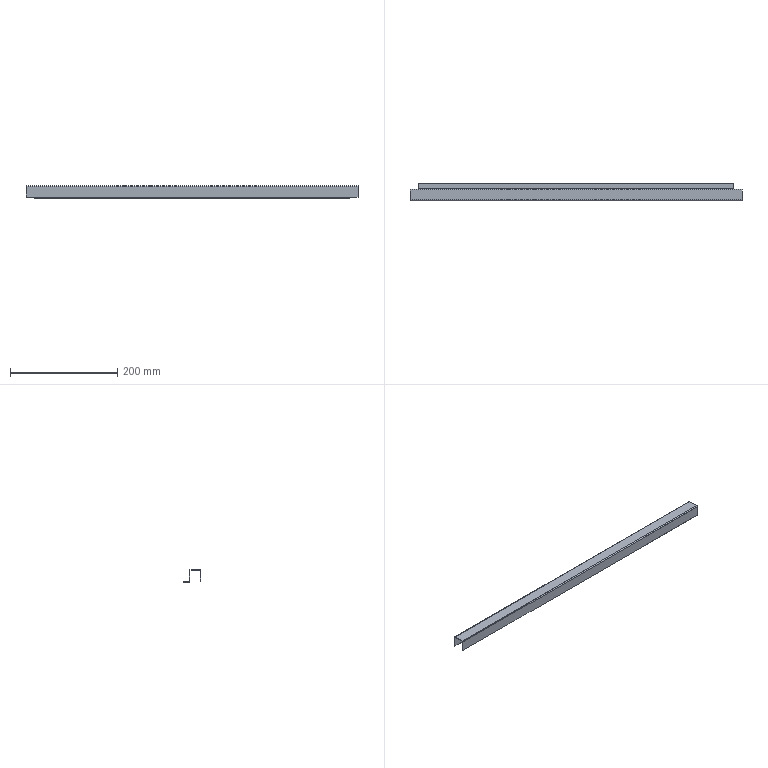Component | SolidWorks | CCQ-1.1-17LowerBeam1-1 | 1 solid | 34 faces | box 620 x 33 x 23 mm | volume 45090 mm3 | plane 24 | cylinder 10 | commonest cylinder face diameters 6 x4 1.473 x3 3.473 x3 | material 304
STEP:
#1=CARTESIAN_POINT('',(-0.2756,-17.185,0.7087));
#2=VERTEX_POINT('',#1);
#3=CARTESIAN_POINT('',(-0.2756,-17.185,0.4724));
#4=VERTEX_POINT('',#3);
#5=CARTESIAN_POINT('',(-0.2756,-17.185,0.5906));
#6=DIRECTION('',(0.,-1.,0.));
#7=DIRECTION('',(0.,0.,-1.));
#8=AXIS2_PLACEMENT_3D('',#5,#6,#7);
#9=CIRCLE('',#8,0.1181);
#10=EDGE_CURVE('',#2,#4,#9,.T.);
#11=ORIENTED_EDGE('',*,*,#10,.T.);
#12=CARTESIAN_POINT('',(-0.2756,-17.146,0.4724));
#13=VERTEX_POINT('',#12);
#14=CARTESIAN_POINT('',(-0.2756,-17.539,0.4724));
#15=DIRECTION('',(0.,1.,0.));
#16=VECTOR('',#15,39.37);
#17=LINE('',#14,#16);
#18=EDGE_CURVE('',#4,#13,#17,.T.);
#19=ORIENTED_EDGE('',*,*,#18,.T.);
#20=CARTESIAN_POINT('',(-0.2756,-17.146,0.7087));
#21=VERTEX_POINT('',#20);
#22=CARTESIAN_POINT('',(-0.2756,-17.146,0.5906));
#23=DIRECTION('',(0.,1.,0.));
#24=DIRECTION('',(0.,0.,-1.));
#25=AXIS2_PLACEMENT_3D('',#22,#23,#24);
#26=CIRCLE('',#25,0.1181);
#27=EDGE_CURVE('',#13,#21,#26,.T.);
#28=ORIENTED_EDGE('',*,*,#27,.T.);
#29=CARTESIAN_POINT('',(-0.2756,-17.539,0.7087));
#30=DIRECTION('',(0.,1.,0.));
#31=VECTOR('',#30,39.37);
#32=LINE('',#29,#31);
#33=EDGE_CURVE('',#2,#21,#32,.T.);
#34=ORIENTED_EDGE('',*,*,#33,.F.);
#35=EDGE_LOOP('',(#11,#19,#28,#34));
#36=FACE_OUTER_BOUND('',#35,.T.);
#37=CARTESIAN_POINT('',(-0.2756,-17.539,0.5906));
#38=DIRECTION('',(0.,1.,0.));
#39=DIRECTION('',(0.,0.,1.));
#40=AXIS2_PLACEMENT_3D('',#37,#38,#39);
#41=CYLINDRICAL_SURFACE('',#40,0.1181);
#42=ADVANCED_FACE('',(#36),#41,.F.);
#43=CARTESIAN_POINT('',(-24.134,-17.185,0.7087));
#44=VERTEX_POINT('',#43);
#45=CARTESIAN_POINT('',(-24.134,-17.185,0.4724));
#46=VERTEX_POINT('',#45);
#47=CARTESIAN_POINT('',(-24.134,-17.185,0.5906));
#48=DIRECTION('',(0.,-1.,0.));
#49=DIRECTION('',(0.,0.,-1.));
#50=AXIS2_PLACEMENT_3D('',#47,#48,#49);
#51=CIRCLE('',#50,0.1181);
#52=EDGE_CURVE('',#44,#46,#51,.T.);
#53=ORIENTED_EDGE('',*,*,#52,.T.);
#54=CARTESIAN_POINT('',(-24.134,-17.146,0.4724));
#55=VERTEX_POINT('',#54);
#56=CARTESIAN_POINT('',(-24.134,-17.539,0.4724));
#57=DIRECTION('',(0.,1.,0.));
#58=VECTOR('',#57,39.37);
#59=LINE('',#56,#58);
#60=EDGE_CURVE('',#46,#55,#59,.T.);
#61=ORIENTED_EDGE('',*,*,#60,.T.);
#62=CARTESIAN_POINT('',(-24.134,-17.146,0.7087));
#63=VERTEX_POINT('',#62);
#64=CARTESIAN_POINT('',(-24.134,-17.146,0.5906));
#65=DIRECTION('',(0.,1.,0.));
#66=DIRECTION('',(0.,0.,1.));
#67=AXIS2_PLACEMENT_3D('',#64,#65,#66);
#68=CIRCLE('',#67,0.1181);
#69=EDGE_CURVE('',#55,#63,#68,.T.);
#70=ORIENTED_EDGE('',*,*,#69,.T.);
#71=CARTESIAN_POINT('',(-24.134,-17.539,0.7087));
#72=DIRECTION('',(0.,1.,0.));
#73=VECTOR('',#72,39.37);
#74=LINE('',#71,#73);
#75=EDGE_CURVE('',#44,#63,#74,.T.);
#76=ORIENTED_EDGE('',*,*,#75,.F.);
#77=EDGE_LOOP('',(#53,#61,#70,#76));
#78=FACE_OUTER_BOUND('',#77,.T.);
#79=CARTESIAN_POINT('',(-24.134,-17.539,0.5906));
#80=DIRECTION('',(0.,1.,0.));
#81=DIRECTION('',(0.,0.,1.));
#82=AXIS2_PLACEMENT_3D('',#79,#80,#81);
#83=CYLINDRICAL_SURFACE('',#82,0.1181);
#84=ADVANCED_FACE('',(#78),#83,.F.);
#85=CARTESIAN_POINT('',(0.,-17.146,-0.04961));
#86=VERTEX_POINT('',#85);
#87=CARTESIAN_POINT('',(0.,-17.185,-0.04961));
#88=VERTEX_POINT('',#87);
#89=CARTESIAN_POINT('',(0.,-17.117,-0.04961));
#90=DIRECTION('',(0.,-1.,0.));
#91=VECTOR('',#90,39.37);
#92=LINE('',#89,#91);
#93=EDGE_CURVE('',#86,#88,#92,.T.);
#94=ORIENTED_EDGE('',*,*,#93,.F.);
#95=CARTESIAN_POINT('',(0.,-17.146,0.719));
#96=VERTEX_POINT('',#95);
#97=CARTESIAN_POINT('',(0.,-17.146,0.748));
#98=DIRECTION('',(0.,0.,1.));
#99=VECTOR('',#98,39.37);
#100=LINE('',#97,#99);
#101=EDGE_CURVE('',#86,#96,#100,.T.);
#102=ORIENTED_EDGE('',*,*,#101,.T.);
#103=CARTESIAN_POINT('',(0.,-17.185,0.719));
#104=VERTEX_POINT('',#103);
#105=CARTESIAN_POINT('',(0.,-17.146,0.719));
#106=DIRECTION('',(0.,-1.,0.));
#107=VECTOR('',#106,39.37);
#108=LINE('',#105,#107);
#109=EDGE_CURVE('',#96,#104,#108,.T.);
#110=ORIENTED_EDGE('',*,*,#109,.T.);
#111=CARTESIAN_POINT('',(0.,-17.185,0.748));
#112=DIRECTION('',(0.,0.,1.));
#113=VECTOR('',#112,39.37);
#114=LINE('',#111,#113);
#115=EDGE_CURVE('',#88,#104,#114,.T.);
#116=ORIENTED_EDGE('',*,*,#115,.F.);
#117=EDGE_LOOP('',(#94,#102,#110,#116));
#118=FACE_OUTER_BOUND('',#117,.T.);
#119=CARTESIAN_POINT('',(0.,-17.117,-0.07874));
#120=DIRECTION('',(1.,0.,0.));
#121=DIRECTION('',(0.,0.,-1.));
#122=AXIS2_PLACEMENT_3D('',#119,#120,#121);
#123=PLANE('',#122);
#124=ADVANCED_FACE('',(#118),#123,.T.);
#125=CARTESIAN_POINT('',(0.,-17.214,0.748));
#126=VERTEX_POINT('',#125);
#127=CARTESIAN_POINT('',(0.,-17.214,0.7874));
#128=VERTEX_POINT('',#127);
#129=CARTESIAN_POINT('',(0.,-17.214,0.748));
#130=DIRECTION('',(0.,0.,1.));
#131=VECTOR('',#130,39.37);
#132=LINE('',#129,#131);
#133=EDGE_CURVE('',#126,#128,#132,.T.);
#134=ORIENTED_EDGE('',*,*,#133,.F.);
#135=CARTESIAN_POINT('',(0.,-17.214,0.719));
#136=DIRECTION('',(1.,0.,0.));
#137=DIRECTION('',(0.,0.,1.));
#138=AXIS2_PLACEMENT_3D('',#135,#136,#137);
#139=CIRCLE('',#138,0.029);
#140=EDGE_CURVE('',#104,#126,#139,.T.);
#141=ORIENTED_EDGE('',*,*,#140,.F.);
#142=ORIENTED_EDGE('',*,*,#109,.F.);
#143=CARTESIAN_POINT('',(0.,-17.214,0.719));
#144=DIRECTION('',(1.,0.,0.));
#145=DIRECTION('',(0.,0.,-1.));
#146=AXIS2_PLACEMENT_3D('',#143,#144,#145);
#147=CIRCLE('',#146,0.06837);
#148=EDGE_CURVE('',#96,#128,#147,.T.);
#149=ORIENTED_EDGE('',*,*,#148,.T.);
#150=EDGE_LOOP('',(#134,#141,#142,#149));
#151=FACE_OUTER_BOUND('',#150,.T.);
#152=CARTESIAN_POINT('',(0.,-17.214,0.748));
#153=DIRECTION('',(1.,0.,0.));
#154=DIRECTION('',(0.,0.,-1.));
#155=AXIS2_PLACEMENT_3D('',#152,#153,#154);
#156=PLANE('',#155);
#157=ADVANCED_FACE('',(#151),#156,.T.);
#158=CARTESIAN_POINT('',(0.,-17.943,0.748));
#159=VERTEX_POINT('',#158);
#160=CARTESIAN_POINT('',(0.,-17.972,0.748));
#161=DIRECTION('',(0.,-1.,0.));
#162=VECTOR('',#161,39.37);
#163=LINE('',#160,#162);
#164=EDGE_CURVE('',#126,#159,#163,.T.);
#165=ORIENTED_EDGE('',*,*,#164,.F.);
#166=ORIENTED_EDGE('',*,*,#133,.T.);
#167=CARTESIAN_POINT('',(0.,-17.943,0.7874));
#168=VERTEX_POINT('',#167);
#169=CARTESIAN_POINT('',(0.,-17.972,0.7874));
#170=DIRECTION('',(0.,-1.,0.));
#171=VECTOR('',#170,39.37);
#172=LINE('',#169,#171);
#173=EDGE_CURVE('',#128,#168,#172,.T.);
#174=ORIENTED_EDGE('',*,*,#173,.T.);
#175=CARTESIAN_POINT('',(0.,-17.943,0.7874));
#176=DIRECTION('',(0.,-0.,-1.));
#177=VECTOR('',#176,39.37);
#178=LINE('',#175,#177);
#179=EDGE_CURVE('',#168,#159,#178,.T.);
#180=ORIENTED_EDGE('',*,*,#179,.T.);
#181=EDGE_LOOP('',(#165,#166,#174,#180));
#182=FACE_OUTER_BOUND('',#181,.T.);
#183=CARTESIAN_POINT('',(0.,-17.146,0.719));
#184=DIRECTION('',(1.,0.,0.));
#185=DIRECTION('',(0.,0.,-1.));
#186=AXIS2_PLACEMENT_3D('',#183,#184,#185);
#187=PLANE('',#186);
#188=ADVANCED_FACE('',(#182),#187,.T.);
#189=CARTESIAN_POINT('',(-24.409,-17.185,0.719));
#190=VERTEX_POINT('',#189);
#191=CARTESIAN_POINT('',(-24.409,-17.146,0.719));
#192=VERTEX_POINT('',#191);
#193=CARTESIAN_POINT('',(-24.409,-17.185,0.719));
#194=DIRECTION('',(0.,1.,-0.));
#195=VECTOR('',#194,39.37);
#196=LINE('',#193,#195);
#197=EDGE_CURVE('',#190,#192,#196,.T.);
#198=ORIENTED_EDGE('',*,*,#197,.F.);
#199=CARTESIAN_POINT('',(-24.409,-17.214,0.748));
#200=VERTEX_POINT('',#199);
#201=CARTESIAN_POINT('',(-24.409,-17.214,0.719));
#202=DIRECTION('',(1.,0.,0.));
#203=DIRECTION('',(0.,0.,1.));
#204=AXIS2_PLACEMENT_3D('',#201,#202,#203);
#205=CIRCLE('',#204,0.029);
#206=EDGE_CURVE('',#190,#200,#205,.T.);
#207=ORIENTED_EDGE('',*,*,#206,.T.);
#208=CARTESIAN_POINT('',(-24.409,-17.214,0.7874));
#209=VERTEX_POINT('',#208);
#210=CARTESIAN_POINT('',(-24.409,-17.214,0.7874));
#211=DIRECTION('',(0.,0.,-1.));
#212=VECTOR('',#211,39.37);
#213=LINE('',#210,#212);
#214=EDGE_CURVE('',#209,#200,#213,.T.);
#215=ORIENTED_EDGE('',*,*,#214,.F.);
#216=CARTESIAN_POINT('',(-24.409,-17.214,0.719));
#217=DIRECTION('',(1.,0.,0.));
#218=DIRECTION('',(0.,0.,-1.));
#219=AXIS2_PLACEMENT_3D('',#216,#217,#218);
#220=CIRCLE('',#219,0.06837);
#221=EDGE_CURVE('',#192,#209,#220,.T.);
#222=ORIENTED_EDGE('',*,*,#221,.F.);
#223=EDGE_LOOP('',(#198,#207,#215,#222));
#224=FACE_OUTER_BOUND('',#223,.T.);
#225=CARTESIAN_POINT('',(-24.409,-17.185,0.719));
#226=DIRECTION('',(-1.,0.,0.));
#227=DIRECTION('',(0.,0.,1.));
#228=AXIS2_PLACEMENT_3D('',#225,#226,#227);
#229=PLANE('',#228);
#230=ADVANCED_FACE('',(#224),#229,.T.);
#231=CARTESIAN_POINT('',(-24.409,-17.185,-0.04961));
#232=VERTEX_POINT('',#231);
#233=CARTESIAN_POINT('',(-24.409,-17.146,-0.04961));
#234=VERTEX_POINT('',#233);
#235=CARTESIAN_POINT('',(-24.409,-17.214,-0.04961));
#236=DIRECTION('',(0.,1.,0.));
#237=VECTOR('',#236,39.37);
#238=LINE('',#235,#237);
#239=EDGE_CURVE('',#232,#234,#238,.T.);
#240=ORIENTED_EDGE('',*,*,#239,.F.);
#241=CARTESIAN_POINT('',(-24.409,-17.185,0.748));
#242=DIRECTION('',(0.,0.,1.));
#243=VECTOR('',#242,39.37);
#244=LINE('',#241,#243);
#245=EDGE_CURVE('',#232,#190,#244,.T.);
#246=ORIENTED_EDGE('',*,*,#245,.T.);
#247=ORIENTED_EDGE('',*,*,#197,.T.);
#248=CARTESIAN_POINT('',(-24.409,-17.146,0.748));
#249=DIRECTION('',(0.,0.,1.));
#250=VECTOR('',#249,39.37);
#251=LINE('',#248,#250);
#252=EDGE_CURVE('',#234,#192,#251,.T.);
#253=ORIENTED_EDGE('',*,*,#252,.F.);
#254=EDGE_LOOP('',(#240,#246,#247,#253));
#255=FACE_OUTER_BOUND('',#254,.T.);
#256=CARTESIAN_POINT('',(-24.409,-17.214,0.7874));
#257=DIRECTION('',(-1.,0.,0.));
#258=DIRECTION('',(0.,0.,1.));
#259=AXIS2_PLACEMENT_3D('',#256,#257,#258);
#260=PLANE('',#259);
#261=ADVANCED_FACE('',(#255),#260,.T.);
#262=CARTESIAN_POINT('',(0.,-17.972,0.719));
#263=VERTEX_POINT('',#262);
#264=CARTESIAN_POINT('',(0.,-18.012,0.719));
#265=VERTEX_POINT('',#264);
#266=CARTESIAN_POINT('',(0.,-17.972,0.719));
#267=DIRECTION('',(0.,-1.,0.));
#268=VECTOR('',#267,39.37);
#269=LINE('',#266,#268);
#270=EDGE_CURVE('',#263,#265,#269,.T.);
#271=ORIENTED_EDGE('',*,*,#270,.F.);
#272=CARTESIAN_POINT('',(0.,-17.943,0.719));
#273=DIRECTION('',(1.,0.,0.));
#274=DIRECTION('',(0.,0.,1.));
#275=AXIS2_PLACEMENT_3D('',#272,#273,#274);
#276=CIRCLE('',#275,0.029);
#277=EDGE_CURVE('',#159,#263,#276,.T.);
#278=ORIENTED_EDGE('',*,*,#277,.F.);
#279=ORIENTED_EDGE('',*,*,#179,.F.);
#280=CARTESIAN_POINT('',(0.,-17.943,0.719));
#281=DIRECTION('',(1.,0.,0.));
#282=DIRECTION('',(0.,0.,-1.));
#283=AXIS2_PLACEMENT_3D('',#280,#281,#282);
#284=CIRCLE('',#283,0.06837);
#285=EDGE_CURVE('',#168,#265,#284,.T.);
#286=ORIENTED_EDGE('',*,*,#285,.T.);
#287=EDGE_LOOP('',(#271,#278,#279,#286));
#288=FACE_OUTER_BOUND('',#287,.T.);
#289=CARTESIAN_POINT('',(0.,-17.972,0.719));
#290=DIRECTION('',(1.,0.,0.));
#291=DIRECTION('',(0.,0.,-1.));
#292=AXIS2_PLACEMENT_3D('',#289,#290,#291);
#293=PLANE('',#292);
#294=ADVANCED_FACE('',(#288),#293,.T.);
#295=CARTESIAN_POINT('',(0.,-17.972,-0.03937));
#296=VERTEX_POINT('',#295);
#297=CARTESIAN_POINT('',(0.,-17.972,0.748));
#298=DIRECTION('',(0.,0.,-1.));
#299=VECTOR('',#298,39.37);
#300=LINE('',#297,#299);
#301=EDGE_CURVE('',#263,#296,#300,.T.);
#302=ORIENTED_EDGE('',*,*,#301,.F.);
#303=ORIENTED_EDGE('',*,*,#270,.T.);
#304=CARTESIAN_POINT('',(0.,-18.012,-0.03937));
#305=VERTEX_POINT('',#304);
#306=CARTESIAN_POINT('',(0.,-18.012,0.748));
#307=DIRECTION('',(0.,0.,-1.));
#308=VECTOR('',#307,39.37);
#309=LINE('',#306,#308);
#310=EDGE_CURVE('',#265,#305,#309,.T.);
#311=ORIENTED_EDGE('',*,*,#310,.T.);
#312=CARTESIAN_POINT('',(0.,-17.972,-0.03937));
#313=DIRECTION('',(0.,-1.,0.));
#314=VECTOR('',#313,39.37);
#315=LINE('',#312,#314);
#316=EDGE_CURVE('',#296,#305,#315,.T.);
#317=ORIENTED_EDGE('',*,*,#316,.F.);
#318=EDGE_LOOP('',(#302,#303,#311,#317));
#319=FACE_OUTER_BOUND('',#318,.T.);
#320=CARTESIAN_POINT('',(0.,-17.943,0.7874));
#321=DIRECTION('',(1.,0.,0.));
#322=DIRECTION('',(0.,0.,-1.));
#323=AXIS2_PLACEMENT_3D('',#320,#321,#322);
#324=PLANE('',#323);
#325=ADVANCED_FACE('',(#319),#324,.T.);
#326=CARTESIAN_POINT('',(-24.409,-17.943,0.748));
#327=VERTEX_POINT('',#326);
#328=CARTESIAN_POINT('',(-24.409,-17.943,0.7874));
#329=VERTEX_POINT('',#328);
#330=CARTESIAN_POINT('',(-24.409,-17.943,0.748));
#331=DIRECTION('',(0.,0.,1.));
#332=VECTOR('',#331,39.37);
#333=LINE('',#330,#332);
#334=EDGE_CURVE('',#327,#329,#333,.T.);
#335=ORIENTED_EDGE('',*,*,#334,.F.);
#336=CARTESIAN_POINT('',(-24.409,-17.972,0.719));
#337=VERTEX_POINT('',#336);
#338=CARTESIAN_POINT('',(-24.409,-17.943,0.719));
#339=DIRECTION('',(1.,0.,0.));
#340=DIRECTION('',(0.,0.,1.));
#341=AXIS2_PLACEMENT_3D('',#338,#339,#340);
#342=CIRCLE('',#341,0.029);
#343=EDGE_CURVE('',#327,#337,#342,.T.);
#344=ORIENTED_EDGE('',*,*,#343,.T.);
#345=CARTESIAN_POINT('',(-24.409,-18.012,0.719));
#346=VERTEX_POINT('',#345);
#347=CARTESIAN_POINT('',(-24.409,-18.012,0.719));
#348=DIRECTION('',(0.,1.,0.));
#349=VECTOR('',#348,39.37);
#350=LINE('',#347,#349);
#351=EDGE_CURVE('',#346,#337,#350,.T.);
#352=ORIENTED_EDGE('',*,*,#351,.F.);
#353=CARTESIAN_POINT('',(-24.409,-17.943,0.719));
#354=DIRECTION('',(1.,0.,0.));
#355=DIRECTION('',(0.,0.,-1.));
#356=AXIS2_PLACEMENT_3D('',#353,#354,#355);
#357=CIRCLE('',#356,0.06837);
#358=EDGE_CURVE('',#329,#346,#357,.T.);
#359=ORIENTED_EDGE('',*,*,#358,.F.);
#360=EDGE_LOOP('',(#335,#344,#352,#359));
#361=FACE_OUTER_BOUND('',#360,.T.);
#362=CARTESIAN_POINT('',(-24.409,-17.943,0.748));
#363=DIRECTION('',(-1.,0.,0.));
#364=DIRECTION('',(0.,0.,1.));
#365=AXIS2_PLACEMENT_3D('',#362,#363,#364);
#366=PLANE('',#365);
#367=ADVANCED_FACE('',(#361),#366,.T.);
#368=CARTESIAN_POINT('',(-24.409,-17.972,0.748));
#369=DIRECTION('',(0.,-1.,0.));
#370=VECTOR('',#369,39.37);
#371=LINE('',#368,#370);
#372=EDGE_CURVE('',#200,#327,#371,.T.);
#373=ORIENTED_EDGE('',*,*,#372,.T.);
#374=ORIENTED_EDGE('',*,*,#334,.T.);
#375=CARTESIAN_POINT('',(-24.409,-17.972,0.7874));
#376=DIRECTION('',(0.,-1.,0.));
#377=VECTOR('',#376,39.37);
#378=LINE('',#375,#377);
#379=EDGE_CURVE('',#209,#329,#378,.T.);
#380=ORIENTED_EDGE('',*,*,#379,.F.);
#381=ORIENTED_EDGE('',*,*,#214,.T.);
#382=EDGE_LOOP('',(#373,#374,#380,#381));
#383=FACE_OUTER_BOUND('',#382,.T.);
#384=CARTESIAN_POINT('',(-24.409,-18.012,0.719));
#385=DIRECTION('',(-1.,0.,0.));
#386=DIRECTION('',(0.,0.,1.));
#387=AXIS2_PLACEMENT_3D('',#384,#385,#386);
#388=PLANE('',#387);
#389=ADVANCED_FACE('',(#383),#388,.T.);
#390=CARTESIAN_POINT('',(-24.409,-18.012,-0.03937));
#391=VERTEX_POINT('',#390);
#392=CARTESIAN_POINT('',(-24.409,-18.012,0.748));
#393=DIRECTION('',(0.,0.,-1.));
#394=VECTOR('',#393,39.37);
#395=LINE('',#392,#394);
#396=EDGE_CURVE('',#346,#391,#395,.T.);
#397=ORIENTED_EDGE('',*,*,#396,.T.);
#398=CARTESIAN_POINT('',(0.,-18.012,-0.03937));
#399=DIRECTION('',(-1.,0.,0.));
#400=VECTOR('',#399,39.37);
#401=LINE('',#398,#400);
#402=EDGE_CURVE('',#305,#391,#401,.T.);
#403=ORIENTED_EDGE('',*,*,#402,.F.);
#404=ORIENTED_EDGE('',*,*,#310,.F.);
#405=CARTESIAN_POINT('',(0.,-18.012,0.719));
#406=DIRECTION('',(-1.,0.,0.));
#407=VECTOR('',#406,39.37);
#408=LINE('',#405,#407);
#409=EDGE_CURVE('',#265,#346,#408,.T.);
#410=ORIENTED_EDGE('',*,*,#409,.T.);
#411=EDGE_LOOP('',(#397,#403,#404,#410));
#412=FACE_OUTER_BOUND('',#411,.T.);
#413=CARTESIAN_POINT('',(0.,-18.012,0.748));
#414=DIRECTION('',(0.,1.,0.));
#415=DIRECTION('',(0.,0.,1.));
#416=AXIS2_PLACEMENT_3D('',#413,#414,#415);
#417=PLANE('',#416);
#418=ADVANCED_FACE('',(#412),#417,.F.);
#419=CARTESIAN_POINT('',(-24.409,-17.972,-0.03937));
#420=VERTEX_POINT('',#419);
#421=CARTESIAN_POINT('',(-24.409,-17.972,-0.03937));
#422=DIRECTION('',(0.,-1.,0.));
#423=VECTOR('',#422,39.37);
#424=LINE('',#421,#423);
#425=EDGE_CURVE('',#420,#391,#424,.T.);
#426=ORIENTED_EDGE('',*,*,#425,.F.);
#427=CARTESIAN_POINT('',(0.,-17.972,-0.03937));
#428=DIRECTION('',(-1.,0.,0.));
#429=VECTOR('',#428,39.37);
#430=LINE('',#427,#429);
#431=EDGE_CURVE('',#296,#420,#430,.T.);
#432=ORIENTED_EDGE('',*,*,#431,.F.);
#433=ORIENTED_EDGE('',*,*,#316,.T.);
#434=ORIENTED_EDGE('',*,*,#402,.T.);
#435=EDGE_LOOP('',(#426,#432,#433,#434));
#436=FACE_OUTER_BOUND('',#435,.T.);
#437=CARTESIAN_POINT('',(0.,-17.972,-0.03937));
#438=DIRECTION('',(0.,0.,-1.));
#439=DIRECTION('',(-1.,0.,0.));
#440=AXIS2_PLACEMENT_3D('',#437,#438,#439);
#441=PLANE('',#440);
#442=ADVANCED_FACE('',(#436),#441,.T.);
#443=CARTESIAN_POINT('',(-24.409,-17.972,0.748));
#444=DIRECTION('',(0.,0.,-1.));
#445=VECTOR('',#444,39.37);
#446=LINE('',#443,#445);
#447=EDGE_CURVE('',#337,#420,#446,.T.);
#448=ORIENTED_EDGE('',*,*,#447,.F.);
#449=CARTESIAN_POINT('',(0.,-17.972,0.719));
#450=DIRECTION('',(-1.,0.,0.));
#451=VECTOR('',#450,39.37);
#452=LINE('',#449,#451);
#453=EDGE_CURVE('',#263,#337,#452,.T.);
#454=ORIENTED_EDGE('',*,*,#453,.F.);
#455=ORIENTED_EDGE('',*,*,#301,.T.);
#456=ORIENTED_EDGE('',*,*,#431,.T.);
#457=EDGE_LOOP('',(#448,#454,#455,#456));
#458=FACE_OUTER_BOUND('',#457,.T.);
#459=CARTESIAN_POINT('',(0.,-17.972,0.748));
#460=DIRECTION('',(0.,1.,0.));
#461=DIRECTION('',(0.,0.,1.));
#462=AXIS2_PLACEMENT_3D('',#459,#460,#461);
#463=PLANE('',#462);
#464=ADVANCED_FACE('',(#458),#463,.T.);
#465=ORIENTED_EDGE('',*,*,#343,.F.);
#466=CARTESIAN_POINT('',(0.,-17.943,0.748));
#467=DIRECTION('',(-1.,0.,0.));
#468=VECTOR('',#467,39.37);
#469=LINE('',#466,#468);
#470=EDGE_CURVE('',#159,#327,#469,.T.);
#471=ORIENTED_EDGE('',*,*,#470,.F.);
#472=ORIENTED_EDGE('',*,*,#277,.T.);
#473=ORIENTED_EDGE('',*,*,#453,.T.);
#474=EDGE_LOOP('',(#465,#471,#472,#473));
#475=FACE_OUTER_BOUND('',#474,.T.);
#476=CARTESIAN_POINT('',(0.,-17.943,0.719));
#477=DIRECTION('',(-1.,0.,0.));
#478=DIRECTION('',(0.,0.,1.));
#479=AXIS2_PLACEMENT_3D('',#476,#477,#478);
#480=CYLINDRICAL_SURFACE('',#479,0.029);
#481=ADVANCED_FACE('',(#475),#480,.F.);
#482=ORIENTED_EDGE('',*,*,#372,.F.);
#483=CARTESIAN_POINT('',(0.,-17.214,0.748));
#484=DIRECTION('',(-1.,0.,0.));
#485=VECTOR('',#484,39.37);
#486=LINE('',#483,#485);
#487=EDGE_CURVE('',#126,#200,#486,.T.);
#488=ORIENTED_EDGE('',*,*,#487,.F.);
#489=ORIENTED_EDGE('',*,*,#164,.T.);
#490=ORIENTED_EDGE('',*,*,#470,.T.);
#491=EDGE_LOOP('',(#482,#488,#489,#490));
#492=FACE_OUTER_BOUND('',#491,.T.);
#493=CARTESIAN_POINT('',(0.,-17.972,0.748));
#494=DIRECTION('',(0.,0.,-1.));
#495=DIRECTION('',(-1.,0.,0.));
#496=AXIS2_PLACEMENT_3D('',#493,#494,#495);
#497=PLANE('',#496);
#498=ADVANCED_FACE('',(#492),#497,.T.);
#499=ORIENTED_EDGE('',*,*,#206,.F.);
#500=CARTESIAN_POINT('',(0.,-17.185,0.719));
#501=DIRECTION('',(-1.,0.,0.));
#502=VECTOR('',#501,39.37);
#503=LINE('',#500,#502);
#504=EDGE_CURVE('',#104,#190,#503,.T.);
#505=ORIENTED_EDGE('',*,*,#504,.F.);
#506=ORIENTED_EDGE('',*,*,#140,.T.);
#507=ORIENTED_EDGE('',*,*,#487,.T.);
#508=EDGE_LOOP('',(#499,#505,#506,#507));
#509=FACE_OUTER_BOUND('',#508,.T.);
#510=CARTESIAN_POINT('',(0.,-17.214,0.719));
#511=DIRECTION('',(-1.,0.,0.));
#512=DIRECTION('',(0.,0.,1.));
#513=AXIS2_PLACEMENT_3D('',#510,#511,#512);
#514=CYLINDRICAL_SURFACE('',#513,0.029);
#515=ADVANCED_FACE('',(#509),#514,.F.);
#516=CARTESIAN_POINT('',(-23.819,-17.185,-0.04961));
#517=VERTEX_POINT('',#516);
#518=CARTESIAN_POINT('',(0.,-17.185,-0.04961));
#519=DIRECTION('',(-1.,0.,0.));
#520=VECTOR('',#519,39.37);
#521=LINE('',#518,#520);
#522=EDGE_CURVE('',#517,#232,#521,.T.);
#523=ORIENTED_EDGE('',*,*,#522,.F.);
#524=CARTESIAN_POINT('',(-23.819,-17.185,-0.04974));
#525=VERTEX_POINT('',#524);
#526=CARTESIAN_POINT('',(-23.819,-17.185,0.748));
#527=DIRECTION('',(0.,0.,1.));
#528=VECTOR('',#527,39.37);
#529=LINE('',#526,#528);
#530=EDGE_CURVE('',#525,#517,#529,.T.);
#531=ORIENTED_EDGE('',*,*,#530,.F.);
#532=CARTESIAN_POINT('',(-0.5906,-17.185,-0.04974));
#533=VERTEX_POINT('',#532);
#534=CARTESIAN_POINT('',(0.,-17.185,-0.04974));
#535=DIRECTION('',(-1.,0.,0.));
#536=VECTOR('',#535,39.37);
#537=LINE('',#534,#536);
#538=EDGE_CURVE('',#533,#525,#537,.T.);
#539=ORIENTED_EDGE('',*,*,#538,.F.);
#540=CARTESIAN_POINT('',(-0.5906,-17.185,-0.04961));
#541=VERTEX_POINT('',#540);
#542=CARTESIAN_POINT('',(-0.5906,-17.185,0.748));
#543=DIRECTION('',(0.,0.,-1.));
#544=VECTOR('',#543,39.37);
#545=LINE('',#542,#544);
#546=EDGE_CURVE('',#541,#533,#545,.T.);
#547=ORIENTED_EDGE('',*,*,#546,.F.);
#548=CARTESIAN_POINT('',(0.,-17.185,-0.04961));
#549=DIRECTION('',(-1.,0.,0.));
#550=VECTOR('',#549,39.37);
#551=LINE('',#548,#550);
#552=EDGE_CURVE('',#88,#541,#551,.T.);
#553=ORIENTED_EDGE('',*,*,#552,.F.);
#554=ORIENTED_EDGE('',*,*,#115,.T.);
#555=ORIENTED_EDGE('',*,*,#504,.T.);
#556=ORIENTED_EDGE('',*,*,#245,.F.);
#557=EDGE_LOOP('',(#523,#531,#539,#547,#553,#554,#555,#556));
#558=FACE_OUTER_BOUND('',#557,.T.);
#559=ORIENTED_EDGE('',*,*,#10,.F.);
#560=CARTESIAN_POINT('',(-0.2756,-17.185,0.5906));
#561=DIRECTION('',(0.,-1.,0.));
#562=DIRECTION('',(0.,0.,-1.));
#563=AXIS2_PLACEMENT_3D('',#560,#561,#562);
#564=CIRCLE('',#563,0.1181);
#565=EDGE_CURVE('',#4,#2,#564,.T.);
#566=ORIENTED_EDGE('',*,*,#565,.F.);
#567=EDGE_LOOP('',(#559,#566));
#568=FACE_BOUND('',#567,.T.);
#569=ORIENTED_EDGE('',*,*,#52,.F.);
#570=CARTESIAN_POINT('',(-24.134,-17.185,0.5906));
#571=DIRECTION('',(0.,-1.,0.));
#572=DIRECTION('',(0.,0.,-1.));
#573=AXIS2_PLACEMENT_3D('',#570,#571,#572);
#574=CIRCLE('',#573,0.1181);
#575=EDGE_CURVE('',#46,#44,#574,.T.);
#576=ORIENTED_EDGE('',*,*,#575,.F.);
#577=EDGE_LOOP('',(#569,#576));
#578=FACE_BOUND('',#577,.T.);
#579=CARTESIAN_POINT('',(0.,-17.185,0.748));
#580=DIRECTION('',(0.,-1.,0.));
#581=DIRECTION('',(0.,0.,-1.));
#582=AXIS2_PLACEMENT_3D('',#579,#580,#581);
#583=PLANE('',#582);
#584=ADVANCED_FACE('',(#558,#568,#578),#583,.T.);
#585=CARTESIAN_POINT('',(-23.819,-17.117,-0.1181));
#586=VERTEX_POINT('',#585);
#587=CARTESIAN_POINT('',(-23.819,-17.117,-0.04974));
#588=DIRECTION('',(-1.,0.,0.));
#589=DIRECTION('',(0.,0.,-1.));
#590=AXIS2_PLACEMENT_3D('',#587,#588,#589);
#591=CIRCLE('',#590,0.06837);
#592=EDGE_CURVE('',#586,#525,#591,.T.);
#593=ORIENTED_EDGE('',*,*,#592,.F.);
#594=CARTESIAN_POINT('',(-0.5906,-17.117,-0.1181));
#595=VERTEX_POINT('',#594);
#596=CARTESIAN_POINT('',(0.,-17.117,-0.1181));
#597=DIRECTION('',(-1.,0.,0.));
#598=VECTOR('',#597,39.37);
#599=LINE('',#596,#598);
#600=EDGE_CURVE('',#595,#586,#599,.T.);
#601=ORIENTED_EDGE('',*,*,#600,.F.);
#602=CARTESIAN_POINT('',(-0.5906,-17.117,-0.04974));
#603=DIRECTION('',(1.,0.,0.));
#604=DIRECTION('',(0.,0.,1.));
#605=AXIS2_PLACEMENT_3D('',#602,#603,#604);
#606=CIRCLE('',#605,0.06837);
#607=EDGE_CURVE('',#533,#595,#606,.T.);
#608=ORIENTED_EDGE('',*,*,#607,.F.);
#609=ORIENTED_EDGE('',*,*,#538,.T.);
#610=EDGE_LOOP('',(#593,#601,#608,#609));
#611=FACE_OUTER_BOUND('',#610,.T.);
#612=CARTESIAN_POINT('',(0.,-17.117,-0.04974));
#613=DIRECTION('',(-1.,0.,0.));
#614=DIRECTION('',(0.,0.,1.));
#615=AXIS2_PLACEMENT_3D('',#612,#613,#614);
#616=CYLINDRICAL_SURFACE('',#615,0.06837);
#617=ADVANCED_FACE('',(#611),#616,.T.);
#618=CARTESIAN_POINT('',(-23.819,-16.713,-0.1181));
#619=VERTEX_POINT('',#618);
#620=CARTESIAN_POINT('',(-23.819,-17.185,-0.1181));
#621=DIRECTION('',(0.,-1.,0.));
#622=VECTOR('',#621,39.37);
#623=LINE('',#620,#622);
#624=EDGE_CURVE('',#619,#586,#623,.T.);
#625=ORIENTED_EDGE('',*,*,#624,.F.);
#626=CARTESIAN_POINT('',(-0.5906,-16.713,-0.1181));
#627=VERTEX_POINT('',#626);
#628=CARTESIAN_POINT('',(0.,-16.713,-0.1181));
#629=DIRECTION('',(-1.,0.,0.));
#630=VECTOR('',#629,39.37);
#631=LINE('',#628,#630);
#632=EDGE_CURVE('',#627,#619,#631,.T.);
#633=ORIENTED_EDGE('',*,*,#632,.F.);
#634=CARTESIAN_POINT('',(-0.5906,-17.185,-0.1181));
#635=DIRECTION('',(0.,1.,0.));
#636=VECTOR('',#635,39.37);
#637=LINE('',#634,#636);
#638=EDGE_CURVE('',#595,#627,#637,.T.);
#639=ORIENTED_EDGE('',*,*,#638,.F.);
#640=ORIENTED_EDGE('',*,*,#600,.T.);
#641=EDGE_LOOP('',(#625,#633,#639,#640));
#642=FACE_OUTER_BOUND('',#641,.T.);
#643=CARTESIAN_POINT('',(0.,-17.185,-0.1181));
#644=DIRECTION('',(0.,0.,-1.));
#645=DIRECTION('',(-1.,0.,0.));
#646=AXIS2_PLACEMENT_3D('',#643,#644,#645);
#647=PLANE('',#646);
#648=ADVANCED_FACE('',(#642),#647,.T.);
#649=CARTESIAN_POINT('',(-23.819,-16.713,-0.07874));
#650=VERTEX_POINT('',#649);
#651=CARTESIAN_POINT('',(-23.819,-16.713,-0.07874));
#652=DIRECTION('',(0.,0.,-1.));
#653=VECTOR('',#652,39.37);
#654=LINE('',#651,#653);
#655=EDGE_CURVE('',#650,#619,#654,.T.);
#656=ORIENTED_EDGE('',*,*,#655,.F.);
#657=CARTESIAN_POINT('',(-0.5906,-16.713,-0.07874));
#658=VERTEX_POINT('',#657);
#659=CARTESIAN_POINT('',(0.,-16.713,-0.07874));
#660=DIRECTION('',(-1.,0.,0.));
#661=VECTOR('',#660,39.37);
#662=LINE('',#659,#661);
#663=EDGE_CURVE('',#658,#650,#662,.T.);
#664=ORIENTED_EDGE('',*,*,#663,.F.);
#665=CARTESIAN_POINT('',(-0.5906,-16.713,-0.07874));
#666=DIRECTION('',(0.,0.,1.));
#667=VECTOR('',#666,39.37);
#668=LINE('',#665,#667);
#669=EDGE_CURVE('',#627,#658,#668,.T.);
#670=ORIENTED_EDGE('',*,*,#669,.F.);
#671=ORIENTED_EDGE('',*,*,#632,.T.);
#672=EDGE_LOOP('',(#656,#664,#670,#671));
#673=FACE_OUTER_BOUND('',#672,.T.);
#674=CARTESIAN_POINT('',(0.,-16.713,-0.07874));
#675=DIRECTION('',(0.,1.,0.));
#676=DIRECTION('',(0.,0.,1.));
#677=AXIS2_PLACEMENT_3D('',#674,#675,#676);
#678=PLANE('',#677);
#679=ADVANCED_FACE('',(#673),#678,.T.);
#680=ORIENTED_EDGE('',*,*,#663,.T.);
#681=CARTESIAN_POINT('',(-23.819,-17.117,-0.07874));
#682=VERTEX_POINT('',#681);
#683=CARTESIAN_POINT('',(-23.819,-17.185,-0.07874));
#684=DIRECTION('',(0.,-1.,0.));
#685=VECTOR('',#684,39.37);
#686=LINE('',#683,#685);
#687=EDGE_CURVE('',#650,#682,#686,.T.);
#688=ORIENTED_EDGE('',*,*,#687,.T.);
#689=CARTESIAN_POINT('',(-0.5906,-17.117,-0.07874));
#690=VERTEX_POINT('',#689);
#691=CARTESIAN_POINT('',(0.,-17.117,-0.07874));
#692=DIRECTION('',(-1.,0.,0.));
#693=VECTOR('',#692,39.37);
#694=LINE('',#691,#693);
#695=EDGE_CURVE('',#690,#682,#694,.T.);
#696=ORIENTED_EDGE('',*,*,#695,.F.);
#697=CARTESIAN_POINT('',(-0.5906,-17.185,-0.07874));
#698=DIRECTION('',(0.,1.,0.));
#699=VECTOR('',#698,39.37);
#700=LINE('',#697,#699);
#701=EDGE_CURVE('',#690,#658,#700,.T.);
#702=ORIENTED_EDGE('',*,*,#701,.T.);
#703=EDGE_LOOP('',(#680,#688,#696,#702));
#704=FACE_OUTER_BOUND('',#703,.T.);
#705=CARTESIAN_POINT('',(0.,-17.185,-0.07874));
#706=DIRECTION('',(0.,0.,-1.));
#707=DIRECTION('',(-1.,0.,0.));
#708=AXIS2_PLACEMENT_3D('',#705,#706,#707);
#709=PLANE('',#708);
#710=ADVANCED_FACE('',(#704),#709,.F.);
#711=ORIENTED_EDGE('',*,*,#695,.T.);
#712=CARTESIAN_POINT('',(-23.819,-17.146,-0.04974));
#713=VERTEX_POINT('',#712);
#714=CARTESIAN_POINT('',(-23.819,-17.117,-0.04974));
#715=DIRECTION('',(-1.,0.,0.));
#716=DIRECTION('',(0.,0.,-1.));
#717=AXIS2_PLACEMENT_3D('',#714,#715,#716);
#718=CIRCLE('',#717,0.029);
#719=EDGE_CURVE('',#682,#713,#718,.T.);
#720=ORIENTED_EDGE('',*,*,#719,.T.);
#721=CARTESIAN_POINT('',(-0.5906,-17.146,-0.04974));
#722=VERTEX_POINT('',#721);
#723=CARTESIAN_POINT('',(0.,-17.146,-0.04974));
#724=DIRECTION('',(-1.,0.,0.));
#725=VECTOR('',#724,39.37);
#726=LINE('',#723,#725);
#727=EDGE_CURVE('',#722,#713,#726,.T.);
#728=ORIENTED_EDGE('',*,*,#727,.F.);
#729=CARTESIAN_POINT('',(-0.5906,-17.117,-0.04974));
#730=DIRECTION('',(1.,0.,0.));
#731=DIRECTION('',(0.,0.,1.));
#732=AXIS2_PLACEMENT_3D('',#729,#730,#731);
#733=CIRCLE('',#732,0.029);
#734=EDGE_CURVE('',#722,#690,#733,.T.);
#735=ORIENTED_EDGE('',*,*,#734,.T.);
#736=EDGE_LOOP('',(#711,#720,#728,#735));
#737=FACE_OUTER_BOUND('',#736,.T.);
#738=CARTESIAN_POINT('',(0.,-17.117,-0.04974));
#739=DIRECTION('',(-1.,0.,0.));
#740=DIRECTION('',(0.,0.,1.));
#741=AXIS2_PLACEMENT_3D('',#738,#739,#740);
#742=CYLINDRICAL_SURFACE('',#741,0.029);
#743=ADVANCED_FACE('',(#737),#742,.F.);
#744=CARTESIAN_POINT('',(-0.2756,-17.146,0.5906));
#745=DIRECTION('',(0.,1.,0.));
#746=DIRECTION('',(0.,0.,-1.));
#747=AXIS2_PLACEMENT_3D('',#744,#745,#746);
#748=CIRCLE('',#747,0.1181);
#749=EDGE_CURVE('',#21,#13,#748,.T.);
#750=ORIENTED_EDGE('',*,*,#749,.F.);
#751=ORIENTED_EDGE('',*,*,#27,.F.);
#752=EDGE_LOOP('',(#750,#751));
#753=FACE_BOUND('',#752,.T.);
#754=CARTESIAN_POINT('',(-24.134,-17.146,0.5906));
#755=DIRECTION('',(0.,1.,0.));
#756=DIRECTION('',(0.,0.,1.));
#757=AXIS2_PLACEMENT_3D('',#754,#755,#756);
#758=CIRCLE('',#757,0.1181);
#759=EDGE_CURVE('',#63,#55,#758,.T.);
#760=ORIENTED_EDGE('',*,*,#759,.F.);
#761=ORIENTED_EDGE('',*,*,#69,.F.);
#762=EDGE_LOOP('',(#760,#761));
#763=FACE_BOUND('',#762,.T.);
#764=CARTESIAN_POINT('',(-23.819,-17.146,-0.04961));
#765=VERTEX_POINT('',#764);
#766=CARTESIAN_POINT('',(-23.819,-17.146,0.748));
#767=DIRECTION('',(0.,0.,1.));
#768=VECTOR('',#767,39.37);
#769=LINE('',#766,#768);
#770=EDGE_CURVE('',#713,#765,#769,.T.);
#771=ORIENTED_EDGE('',*,*,#770,.T.);
#772=CARTESIAN_POINT('',(0.,-17.146,-0.04961));
#773=DIRECTION('',(-1.,0.,0.));
#774=VECTOR('',#773,39.37);
#775=LINE('',#772,#774);
#776=EDGE_CURVE('',#765,#234,#775,.T.);
#777=ORIENTED_EDGE('',*,*,#776,.T.);
#778=ORIENTED_EDGE('',*,*,#252,.T.);
#779=CARTESIAN_POINT('',(0.,-17.146,0.719));
#780=DIRECTION('',(-1.,0.,0.));
#781=VECTOR('',#780,39.37);
#782=LINE('',#779,#781);
#783=EDGE_CURVE('',#96,#192,#782,.T.);
#784=ORIENTED_EDGE('',*,*,#783,.F.);
#785=ORIENTED_EDGE('',*,*,#101,.F.);
#786=CARTESIAN_POINT('',(-0.5906,-17.146,-0.04961));
#787=VERTEX_POINT('',#786);
#788=CARTESIAN_POINT('',(0.,-17.146,-0.04961));
#789=DIRECTION('',(-1.,0.,0.));
#790=VECTOR('',#789,39.37);
#791=LINE('',#788,#790);
#792=EDGE_CURVE('',#86,#787,#791,.T.);
#793=ORIENTED_EDGE('',*,*,#792,.T.);
#794=CARTESIAN_POINT('',(-0.5906,-17.146,0.748));
#795=DIRECTION('',(0.,0.,-1.));
#796=VECTOR('',#795,39.37);
#797=LINE('',#794,#796);
#798=EDGE_CURVE('',#787,#722,#797,.T.);
#799=ORIENTED_EDGE('',*,*,#798,.T.);
#800=ORIENTED_EDGE('',*,*,#727,.T.);
#801=EDGE_LOOP('',(#771,#777,#778,#784,#785,#793,#799,#800));
#802=FACE_OUTER_BOUND('',#801,.T.);
#803=CARTESIAN_POINT('',(0.,-17.146,0.748));
#804=DIRECTION('',(0.,-1.,0.));
#805=DIRECTION('',(0.,0.,-1.));
#806=AXIS2_PLACEMENT_3D('',#803,#804,#805);
#807=PLANE('',#806);
#808=ADVANCED_FACE('',(#753,#763,#802),#807,.F.);
#809=ORIENTED_EDGE('',*,*,#221,.T.);
#810=CARTESIAN_POINT('',(0.,-17.214,0.7874));
#811=DIRECTION('',(-1.,0.,0.));
#812=VECTOR('',#811,39.37);
#813=LINE('',#810,#812);
#814=EDGE_CURVE('',#128,#209,#813,.T.);
#815=ORIENTED_EDGE('',*,*,#814,.F.);
#816=ORIENTED_EDGE('',*,*,#148,.F.);
#817=ORIENTED_EDGE('',*,*,#783,.T.);
#818=EDGE_LOOP('',(#809,#815,#816,#817));
#819=FACE_OUTER_BOUND('',#818,.T.);
#820=CARTESIAN_POINT('',(0.,-17.214,0.719));
#821=DIRECTION('',(-1.,0.,0.));
#822=DIRECTION('',(0.,0.,1.));
#823=AXIS2_PLACEMENT_3D('',#820,#821,#822);
#824=CYLINDRICAL_SURFACE('',#823,0.06837);
#825=ADVANCED_FACE('',(#819),#824,.T.);
#826=ORIENTED_EDGE('',*,*,#379,.T.);
#827=CARTESIAN_POINT('',(0.,-17.943,0.7874));
#828=DIRECTION('',(-1.,0.,0.));
#829=VECTOR('',#828,39.37);
#830=LINE('',#827,#829);
#831=EDGE_CURVE('',#168,#329,#830,.T.);
#832=ORIENTED_EDGE('',*,*,#831,.F.);
#833=ORIENTED_EDGE('',*,*,#173,.F.);
#834=ORIENTED_EDGE('',*,*,#814,.T.);
#835=EDGE_LOOP('',(#826,#832,#833,#834));
#836=FACE_OUTER_BOUND('',#835,.T.);
#837=CARTESIAN_POINT('',(0.,-17.972,0.7874));
#838=DIRECTION('',(0.,0.,-1.));
#839=DIRECTION('',(-1.,0.,0.));
#840=AXIS2_PLACEMENT_3D('',#837,#838,#839);
#841=PLANE('',#840);
#842=ADVANCED_FACE('',(#836),#841,.F.);
#843=ORIENTED_EDGE('',*,*,#358,.T.);
#844=ORIENTED_EDGE('',*,*,#409,.F.);
#845=ORIENTED_EDGE('',*,*,#285,.F.);
#846=ORIENTED_EDGE('',*,*,#831,.T.);
#847=EDGE_LOOP('',(#843,#844,#845,#846));
#848=FACE_OUTER_BOUND('',#847,.T.);
#849=CARTESIAN_POINT('',(0.,-17.943,0.719));
#850=DIRECTION('',(-1.,0.,0.));
#851=DIRECTION('',(0.,0.,1.));
#852=AXIS2_PLACEMENT_3D('',#849,#850,#851);
#853=CYLINDRICAL_SURFACE('',#852,0.06837);
#854=ADVANCED_FACE('',(#848),#853,.T.);
#855=ORIENTED_EDGE('',*,*,#396,.F.);
#856=ORIENTED_EDGE('',*,*,#351,.T.);
#857=ORIENTED_EDGE('',*,*,#447,.T.);
#858=ORIENTED_EDGE('',*,*,#425,.T.);
#859=EDGE_LOOP('',(#855,#856,#857,#858));
#860=FACE_OUTER_BOUND('',#859,.T.);
#861=CARTESIAN_POINT('',(-24.409,-17.943,0.719));
#862=DIRECTION('',(-1.,0.,0.));
#863=DIRECTION('',(0.,0.,1.));
#864=AXIS2_PLACEMENT_3D('',#861,#862,#863);
#865=PLANE('',#864);
#866=ADVANCED_FACE('',(#860),#865,.T.);
#867=ORIENTED_EDGE('',*,*,#60,.F.);
#868=ORIENTED_EDGE('',*,*,#575,.T.);
#869=ORIENTED_EDGE('',*,*,#75,.T.);
#870=ORIENTED_EDGE('',*,*,#759,.T.);
#871=EDGE_LOOP('',(#867,#868,#869,#870));
#872=FACE_OUTER_BOUND('',#871,.T.);
#873=CARTESIAN_POINT('',(-24.134,-17.539,0.5906));
#874=DIRECTION('',(0.,1.,0.));
#875=DIRECTION('',(0.,0.,1.));
#876=AXIS2_PLACEMENT_3D('',#873,#874,#875);
#877=CYLINDRICAL_SURFACE('',#876,0.1181);
#878=ADVANCED_FACE('',(#872),#877,.F.);
#879=ORIENTED_EDGE('',*,*,#18,.F.);
#880=ORIENTED_EDGE('',*,*,#565,.T.);
#881=ORIENTED_EDGE('',*,*,#33,.T.);
#882=ORIENTED_EDGE('',*,*,#749,.T.);
#883=EDGE_LOOP('',(#879,#880,#881,#882));
#884=FACE_OUTER_BOUND('',#883,.T.);
#885=CARTESIAN_POINT('',(-0.2756,-17.539,0.5906));
#886=DIRECTION('',(0.,1.,0.));
#887=DIRECTION('',(0.,0.,1.));
#888=AXIS2_PLACEMENT_3D('',#885,#886,#887);
#889=CYLINDRICAL_SURFACE('',#888,0.1181);
#890=ADVANCED_FACE('',(#884),#889,.F.);
#891=ORIENTED_EDGE('',*,*,#552,.T.);
#892=CARTESIAN_POINT('',(-0.5906,-16.949,-0.04961));
#893=DIRECTION('',(0.,1.,0.));
#894=VECTOR('',#893,39.37);
#895=LINE('',#892,#894);
#896=EDGE_CURVE('',#541,#787,#895,.T.);
#897=ORIENTED_EDGE('',*,*,#896,.T.);
#898=ORIENTED_EDGE('',*,*,#792,.F.);
#899=ORIENTED_EDGE('',*,*,#93,.T.);
#900=EDGE_LOOP('',(#891,#897,#898,#899));
#901=FACE_OUTER_BOUND('',#900,.T.);
#902=CARTESIAN_POINT('',(-0.2933,-16.949,-0.04961));
#903=DIRECTION('',(0.,0.,1.));
#904=DIRECTION('',(1.,0.,0.));
#905=AXIS2_PLACEMENT_3D('',#902,#903,#904);
#906=PLANE('',#905);
#907=ADVANCED_FACE('',(#901),#906,.F.);
#908=ORIENTED_EDGE('',*,*,#546,.T.);
#909=ORIENTED_EDGE('',*,*,#607,.T.);
#910=ORIENTED_EDGE('',*,*,#638,.T.);
#911=ORIENTED_EDGE('',*,*,#669,.T.);
#912=ORIENTED_EDGE('',*,*,#701,.F.);
#913=ORIENTED_EDGE('',*,*,#734,.F.);
#914=ORIENTED_EDGE('',*,*,#798,.F.);
#915=ORIENTED_EDGE('',*,*,#896,.F.);
#916=EDGE_LOOP('',(#908,#909,#910,#911,#912,#913,#914,#915));
#917=FACE_OUTER_BOUND('',#916,.T.);
#918=CARTESIAN_POINT('',(-0.5906,-16.949,-0.122));
#919=DIRECTION('',(-1.,0.,0.));
#920=DIRECTION('',(0.,0.,1.));
#921=AXIS2_PLACEMENT_3D('',#918,#919,#920);
#922=PLANE('',#921);
#923=ADVANCED_FACE('',(#917),#922,.F.);
#924=ORIENTED_EDGE('',*,*,#522,.T.);
#925=ORIENTED_EDGE('',*,*,#239,.T.);
#926=ORIENTED_EDGE('',*,*,#776,.F.);
#927=CARTESIAN_POINT('',(-23.819,-16.949,-0.04961));
#928=DIRECTION('',(0.,-1.,0.));
#929=VECTOR('',#928,39.37);
#930=LINE('',#927,#929);
#931=EDGE_CURVE('',#765,#517,#930,.T.);
#932=ORIENTED_EDGE('',*,*,#931,.T.);
#933=EDGE_LOOP('',(#924,#925,#926,#932));
#934=FACE_OUTER_BOUND('',#933,.T.);
#935=CARTESIAN_POINT('',(-24.116,-16.949,-0.04961));
#936=DIRECTION('',(0.,0.,1.));
#937=DIRECTION('',(1.,0.,0.));
#938=AXIS2_PLACEMENT_3D('',#935,#936,#937);
#939=PLANE('',#938);
#940=ADVANCED_FACE('',(#934),#939,.F.);
#941=ORIENTED_EDGE('',*,*,#530,.T.);
#942=ORIENTED_EDGE('',*,*,#931,.F.);
#943=ORIENTED_EDGE('',*,*,#770,.F.);
#944=ORIENTED_EDGE('',*,*,#719,.F.);
#945=ORIENTED_EDGE('',*,*,#687,.F.);
#946=ORIENTED_EDGE('',*,*,#655,.T.);
#947=ORIENTED_EDGE('',*,*,#624,.T.);
#948=ORIENTED_EDGE('',*,*,#592,.T.);
#949=EDGE_LOOP('',(#941,#942,#943,#944,#945,#946,#947,#948));
#950=FACE_OUTER_BOUND('',#949,.T.);
#951=CARTESIAN_POINT('',(-23.819,-16.949,-0.122));
#952=DIRECTION('',(1.,0.,0.));
#953=DIRECTION('',(0.,0.,-1.));
#954=AXIS2_PLACEMENT_3D('',#951,#952,#953);
#955=PLANE('',#954);
#956=ADVANCED_FACE('',(#950),#955,.F.);
#957=CLOSED_SHELL('',(#42,#84,#124,#157,#188,#230,#261,#294,#325,#367,#389,#418,#442,#464,#481,#498,#515,#584,#617,#648,#679,#710,#743,#808,#825,#842,#854,#866,#878,#890,#907,#923,#940,#956));
#958=MANIFOLD_SOLID_BREP('',#957);
#959=CARTESIAN_POINT('',(0.,0.,0.));
#960=DIRECTION('',(0.,0.,1.));
#961=DIRECTION('',(1.,0.,0.));
#962=AXIS2_PLACEMENT_3D('',#959,#960,#961);
#963=(LENGTH_UNIT()NAMED_UNIT(*)SI_UNIT($,.METRE.));
#964=LENGTH_MEASURE_WITH_UNIT(LENGTH_MEASURE(0.0254),#963);
#965=DIMENSIONAL_EXPONENTS(1.,0.,0.,0.,0.,0.,0.);
#966=(CONVERSION_BASED_UNIT('',#964)LENGTH_UNIT()NAMED_UNIT(#965));
#967=UNCERTAINTY_MEASURE_WITH_UNIT(LENGTH_MEASURE(0.00001),#966,'','');
#968=(NAMED_UNIT(*)PLANE_ANGLE_UNIT()SI_UNIT($,.RADIAN.));
#969=(NAMED_UNIT(*)SI_UNIT($,.STERADIAN.)SOLID_ANGLE_UNIT());
#970=(GEOMETRIC_REPRESENTATION_CONTEXT(3)GLOBAL_UNCERTAINTY_ASSIGNED_CONTEXT((#967))GLOBAL_UNIT_ASSIGNED_CONTEXT((#966,#968,#969))REPRESENTATION_CONTEXT('',''));
#971=ADVANCED_BREP_SHAPE_REPRESENTATION('',(#958,#962),#970);
#972=COLOUR_RGB('',0.7922,0.8196,0.9333);
#973=FILL_AREA_STYLE_COLOUR('',#972);
#974=FILL_AREA_STYLE('',(#973));
#975=SURFACE_STYLE_FILL_AREA(#974);
#976=SURFACE_SIDE_STYLE('',(#975));
#977=SURFACE_STYLE_USAGE(.BOTH.,#976);
#978=PRESENTATION_STYLE_ASSIGNMENT((#977));
#979=STYLED_ITEM('',(#978),#958);
#980=PRESENTATION_LAYER_ASSIGNMENT('','',(#979));
#981=(LENGTH_UNIT()NAMED_UNIT(*)SI_UNIT($,.METRE.));
#982=LENGTH_MEASURE_WITH_UNIT(LENGTH_MEASURE(0.0254),#981);
#983=DIMENSIONAL_EXPONENTS(1.,0.,0.,0.,0.,0.,0.);
#984=(CONVERSION_BASED_UNIT('',#982)LENGTH_UNIT()NAMED_UNIT(#983));
#985=UNCERTAINTY_MEASURE_WITH_UNIT(LENGTH_MEASURE(0.00001),#984,'','');
#986=(NAMED_UNIT(*)PLANE_ANGLE_UNIT()SI_UNIT($,.RADIAN.));
#987=(NAMED_UNIT(*)SI_UNIT($,.STERADIAN.)SOLID_ANGLE_UNIT());
#988=(GEOMETRIC_REPRESENTATION_CONTEXT(3)GLOBAL_UNCERTAINTY_ASSIGNED_CONTEXT((#985))GLOBAL_UNIT_ASSIGNED_CONTEXT((#984,#986,#987))REPRESENTATION_CONTEXT('',''));
#989=MECHANICAL_DESIGN_GEOMETRIC_PRESENTATION_REPRESENTATION('',(#979),#988);